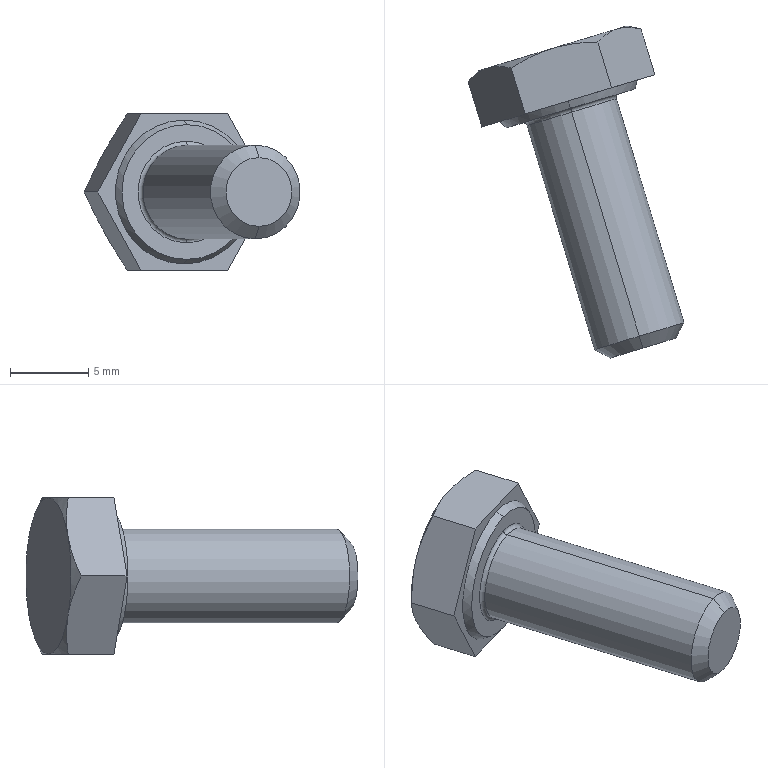Component | SolidWorks | GB_T5781-2000[HexHeadBoltFullThreadGradeCM6_16]-1 | 1 solid | 24 faces | box 13.82 x 21.23 x 10 mm | volume 780 mm3 | cone 10 | plane 10 | cylinder 2 | torus 2 | commonest cylinder face diameters 6 x2
STEP:
#1=COLOUR_RGB('',0.7922,0.8196,0.9333);
#2=FILL_AREA_STYLE_COLOUR('',#1);
#3=FILL_AREA_STYLE('',(#2));
#4=SURFACE_STYLE_FILL_AREA(#3);
#5=SURFACE_SIDE_STYLE('',(#4));
#6=SURFACE_STYLE_USAGE(.BOTH.,#5);
#7=PRESENTATION_STYLE_ASSIGNMENT((#6));
#8=CARTESIAN_POINT('',(-9.837,5.616,-1.85));
#9=VERTEX_POINT('',#8);
#10=CARTESIAN_POINT('',(-9.837,5.616,-2.087));
#11=VERTEX_POINT('',#10);
#12=CARTESIAN_POINT('',(-9.837,5.616,-1.969));
#13=DIRECTION('',(-0.2889,0.9574,0.));
#14=DIRECTION('',(0.,0.,1.));
#15=AXIS2_PLACEMENT_3D('',#12,#13,#14);
#16=CIRCLE('',#15,0.1181);
#17=EDGE_CURVE('',#9,#11,#16,.T.);
#18=ORIENTED_EDGE('',*,*,#17,.F.);
#19=CARTESIAN_POINT('',(-9.667,5.053,-1.85));
#20=VERTEX_POINT('',#19);
#21=CARTESIAN_POINT('',(-9.885,5.776,-1.85));
#22=DIRECTION('',(0.2889,-0.9574,0.));
#23=VECTOR('',#22,39.37);
#24=LINE('',#21,#23);
#25=EDGE_CURVE('',#9,#20,#24,.T.);
#26=ORIENTED_EDGE('',*,*,#25,.T.);
#27=CARTESIAN_POINT('',(-9.667,5.053,-2.087));
#28=VERTEX_POINT('',#27);
#29=CARTESIAN_POINT('',(-9.667,5.053,-1.969));
#30=DIRECTION('',(-0.2889,0.9574,0.));
#31=DIRECTION('',(0.,0.,-1.));
#32=AXIS2_PLACEMENT_3D('',#29,#30,#31);
#33=CIRCLE('',#32,0.1181);
#34=EDGE_CURVE('',#20,#28,#33,.T.);
#35=ORIENTED_EDGE('',*,*,#34,.T.);
#36=CARTESIAN_POINT('',(-9.885,5.776,-2.087));
#37=DIRECTION('',(0.2889,-0.9574,0.));
#38=VECTOR('',#37,39.37);
#39=LINE('',#36,#38);
#40=EDGE_CURVE('',#11,#28,#39,.T.);
#41=ORIENTED_EDGE('',*,*,#40,.F.);
#42=EDGE_LOOP('',(#18,#26,#35,#41));
#43=FACE_OUTER_BOUND('',#42,.T.);
#44=CARTESIAN_POINT('',(-9.885,5.776,-1.969));
#45=DIRECTION('',(0.2889,-0.9574,0.));
#46=DIRECTION('',(0.,0.,-1.));
#47=AXIS2_PLACEMENT_3D('',#44,#45,#46);
#48=CYLINDRICAL_SURFACE('',#47,0.1181);
#49=ADVANCED_FACE('',(#43),#48,.T.);
#50=CARTESIAN_POINT('',(-9.658,5.022,-2.055));
#51=VERTEX_POINT('',#50);
#52=CARTESIAN_POINT('',(-9.658,5.022,-1.882));
#53=VERTEX_POINT('',#52);
#54=CARTESIAN_POINT('',(-9.658,5.022,-1.969));
#55=DIRECTION('',(0.2889,-0.9574,0.));
#56=DIRECTION('',(0.,0.,-1.));
#57=AXIS2_PLACEMENT_3D('',#54,#55,#56);
#58=CIRCLE('',#57,0.08661);
#59=EDGE_CURVE('',#51,#53,#58,.T.);
#60=ORIENTED_EDGE('',*,*,#59,.F.);
#61=CARTESIAN_POINT('',(-9.658,5.022,-2.055));
#62=DIRECTION('',(-0.2043,0.677,-0.7071));
#63=VECTOR('',#62,39.37);
#64=LINE('',#61,#63);
#65=EDGE_CURVE('',#51,#28,#64,.T.);
#66=ORIENTED_EDGE('',*,*,#65,.T.);
#67=ORIENTED_EDGE('',*,*,#34,.F.);
#68=CARTESIAN_POINT('',(-9.658,5.022,-1.882));
#69=DIRECTION('',(-0.2043,0.677,0.7071));
#70=VECTOR('',#69,39.37);
#71=LINE('',#68,#70);
#72=EDGE_CURVE('',#53,#20,#71,.T.);
#73=ORIENTED_EDGE('',*,*,#72,.F.);
#74=EDGE_LOOP('',(#60,#66,#67,#73));
#75=FACE_OUTER_BOUND('',#74,.T.);
#76=CARTESIAN_POINT('',(-9.658,5.022,-1.969));
#77=DIRECTION('',(-0.2889,0.9574,0.));
#78=DIRECTION('',(0.,0.,1.));
#79=AXIS2_PLACEMENT_3D('',#76,#77,#78);
#80=CONICAL_SURFACE('',#79,0.08661,0.7854);
#81=ADVANCED_FACE('',(#75),#80,.T.);
#82=CARTESIAN_POINT('',(-9.84,5.626,-2.096));
#83=VERTEX_POINT('',#82);
#84=CARTESIAN_POINT('',(-9.84,5.626,-1.841));
#85=VERTEX_POINT('',#84);
#86=CARTESIAN_POINT('',(-9.84,5.626,-1.969));
#87=DIRECTION('',(-0.2889,0.9574,0.));
#88=DIRECTION('',(0.,0.,1.));
#89=AXIS2_PLACEMENT_3D('',#86,#87,#88);
#90=CIRCLE('',#89,0.128);
#91=EDGE_CURVE('',#83,#85,#90,.T.);
#92=ORIENTED_EDGE('',*,*,#91,.F.);
#93=CARTESIAN_POINT('',(-9.837,5.616,-2.096));
#94=DIRECTION('',(0.9574,0.2889,0.));
#95=DIRECTION('',(-0.2889,0.9574,0.));
#96=AXIS2_PLACEMENT_3D('',#93,#94,#95);
#97=CIRCLE('',#96,0.009843);
#98=EDGE_CURVE('',#83,#11,#97,.T.);
#99=ORIENTED_EDGE('',*,*,#98,.T.);
#100=CARTESIAN_POINT('',(-9.837,5.616,-1.969));
#101=DIRECTION('',(-0.2889,0.9574,0.));
#102=DIRECTION('',(0.,0.,1.));
#103=AXIS2_PLACEMENT_3D('',#100,#101,#102);
#104=CIRCLE('',#103,0.1181);
#105=EDGE_CURVE('',#11,#9,#104,.T.);
#106=ORIENTED_EDGE('',*,*,#105,.T.);
#107=CARTESIAN_POINT('',(-9.837,5.616,-1.841));
#108=DIRECTION('',(-0.9574,-0.2889,0.));
#109=DIRECTION('',(0.2889,-0.9574,0.));
#110=AXIS2_PLACEMENT_3D('',#107,#108,#109);
#111=CIRCLE('',#110,0.009843);
#112=EDGE_CURVE('',#85,#9,#111,.T.);
#113=ORIENTED_EDGE('',*,*,#112,.F.);
#114=EDGE_LOOP('',(#92,#99,#106,#113));
#115=FACE_OUTER_BOUND('',#114,.T.);
#116=CARTESIAN_POINT('',(-9.837,5.616,-1.969));
#117=DIRECTION('',(-0.2889,0.9574,0.));
#118=DIRECTION('',(0.,0.,1.));
#119=AXIS2_PLACEMENT_3D('',#116,#117,#118);
#120=TOROIDAL_SURFACE('',#119,0.128,0.009843);
#121=ADVANCED_FACE('',(#115),#120,.F.);
#122=CARTESIAN_POINT('',(-9.84,5.626,-1.799));
#123=VERTEX_POINT('',#122);
#124=CARTESIAN_POINT('',(-9.84,5.626,-2.138));
#125=VERTEX_POINT('',#124);
#126=CARTESIAN_POINT('',(-9.84,5.626,-1.969));
#127=DIRECTION('',(-0.2889,0.9574,0.));
#128=DIRECTION('',(0.,0.,1.));
#129=AXIS2_PLACEMENT_3D('',#126,#127,#128);
#130=CIRCLE('',#129,0.1698);
#131=EDGE_CURVE('',#123,#125,#130,.T.);
#132=ORIENTED_EDGE('',*,*,#131,.T.);
#133=CARTESIAN_POINT('',(-9.846,5.644,-2.15));
#134=VERTEX_POINT('',#133);
#135=CARTESIAN_POINT('',(-9.846,5.644,-2.15));
#136=DIRECTION('',(-0.2502,0.8291,-0.5));
#137=VECTOR('',#136,39.37);
#138=LINE('',#135,#137);
#139=EDGE_CURVE('',#125,#134,#138,.T.);
#140=ORIENTED_EDGE('',*,*,#139,.T.);
#141=CARTESIAN_POINT('',(-9.846,5.644,-1.787));
#142=VERTEX_POINT('',#141);
#143=CARTESIAN_POINT('',(-9.846,5.644,-1.969));
#144=DIRECTION('',(-0.2889,0.9574,0.));
#145=DIRECTION('',(0.,0.,1.));
#146=AXIS2_PLACEMENT_3D('',#143,#144,#145);
#147=CIRCLE('',#146,0.1811);
#148=EDGE_CURVE('',#142,#134,#147,.T.);
#149=ORIENTED_EDGE('',*,*,#148,.F.);
#150=CARTESIAN_POINT('',(-9.846,5.644,-1.787));
#151=DIRECTION('',(-0.2502,0.8291,0.5));
#152=VECTOR('',#151,39.37);
#153=LINE('',#150,#152);
#154=EDGE_CURVE('',#123,#142,#153,.T.);
#155=ORIENTED_EDGE('',*,*,#154,.F.);
#156=EDGE_LOOP('',(#132,#140,#149,#155));
#157=FACE_OUTER_BOUND('',#156,.T.);
#158=CARTESIAN_POINT('',(-9.846,5.644,-1.969));
#159=DIRECTION('',(-0.2889,0.9574,0.));
#160=DIRECTION('',(0.,0.,1.));
#161=AXIS2_PLACEMENT_3D('',#158,#159,#160);
#162=CONICAL_SURFACE('',#161,0.1811,0.5236);
#163=ADVANCED_FACE('',(#157),#162,.T.);
#164=ORIENTED_EDGE('',*,*,#131,.F.);
#165=CARTESIAN_POINT('',(-9.84,5.626,-1.969));
#166=DIRECTION('',(-0.2889,0.9574,0.));
#167=DIRECTION('',(0.,0.,1.));
#168=AXIS2_PLACEMENT_3D('',#165,#166,#167);
#169=CIRCLE('',#168,0.1698);
#170=EDGE_CURVE('',#125,#123,#169,.T.);
#171=ORIENTED_EDGE('',*,*,#170,.F.);
#172=EDGE_LOOP('',(#164,#171));
#173=FACE_OUTER_BOUND('',#172,.T.);
#174=CARTESIAN_POINT('',(-9.84,5.626,-1.969));
#175=DIRECTION('',(-0.2889,0.9574,0.));
#176=DIRECTION('',(0.,0.,1.));
#177=AXIS2_PLACEMENT_3D('',#174,#175,#176);
#178=CIRCLE('',#177,0.128);
#179=EDGE_CURVE('',#85,#83,#178,.T.);
#180=ORIENTED_EDGE('',*,*,#179,.T.);
#181=ORIENTED_EDGE('',*,*,#91,.T.);
#182=EDGE_LOOP('',(#180,#181));
#183=FACE_BOUND('',#182,.T.);
#184=CARTESIAN_POINT('',(-9.622,5.691,-1.969));
#185=DIRECTION('',(0.2889,-0.9574,0.));
#186=DIRECTION('',(0.,0.,-1.));
#187=AXIS2_PLACEMENT_3D('',#184,#185,#186);
#188=PLANE('',#187);
#189=ADVANCED_FACE('',(#173,#183),#188,.T.);
#190=CARTESIAN_POINT('',(-9.737,5.677,-2.165));
#191=VERTEX_POINT('',#190);
#192=CARTESIAN_POINT('',(-9.628,5.71,-1.969));
#193=VERTEX_POINT('',#192);
#194=CARTESIAN_POINT('',(-9.737,5.677,-2.165));
#195=DIRECTION('',(0.4787,0.1444,0.866));
#196=VECTOR('',#195,39.37);
#197=LINE('',#194,#196);
#198=EDGE_CURVE('',#191,#193,#197,.T.);
#199=ORIENTED_EDGE('',*,*,#198,.F.);
#200=CARTESIAN_POINT('',(-9.772,5.792,-2.165));
#201=VERTEX_POINT('',#200);
#202=CARTESIAN_POINT('',(-9.731,5.658,-2.165));
#203=DIRECTION('',(-0.2889,0.9574,0.));
#204=VECTOR('',#203,39.37);
#205=LINE('',#202,#204);
#206=EDGE_CURVE('',#191,#201,#205,.T.);
#207=ORIENTED_EDGE('',*,*,#206,.T.);
#208=CARTESIAN_POINT('',(-9.722,5.826,-2.067));
#209=VERTEX_POINT('',#208);
#210=CARTESIAN_POINT('',(-9.722,5.826,-2.067));
#211=CARTESIAN_POINT('',(-9.727,5.824,-2.075));
#212=CARTESIAN_POINT('',(-9.731,5.822,-2.084));
#213=CARTESIAN_POINT('',(-9.74,5.818,-2.1));
#214=CARTESIAN_POINT('',(-9.744,5.816,-2.109));
#215=CARTESIAN_POINT('',(-9.757,5.807,-2.133));
#216=CARTESIAN_POINT('',(-9.764,5.8,-2.149));
#217=CARTESIAN_POINT('',(-9.772,5.792,-2.165));
#218=B_SPLINE_CURVE_WITH_KNOTS('',3,(#210,#211,#212,#213,#214,#215,#216,#217),.UNSPECIFIED.,.F.,.F.,(4,2,2,4),(0.002921,0.003649,0.004376,0.005831),.UNSPECIFIED.);
#219=EDGE_CURVE('',#209,#201,#218,.T.);
#220=ORIENTED_EDGE('',*,*,#219,.F.);
#221=CARTESIAN_POINT('',(-9.663,5.825,-1.969));
#222=VERTEX_POINT('',#221);
#223=CARTESIAN_POINT('',(-9.663,5.825,-1.969));
#224=CARTESIAN_POINT('',(-9.684,5.83,-2.001));
#225=CARTESIAN_POINT('',(-9.704,5.831,-2.033));
#226=CARTESIAN_POINT('',(-9.722,5.826,-2.067));
#227=B_SPLINE_CURVE_WITH_KNOTS('',3,(#223,#224,#225,#226),.UNSPECIFIED.,.F.,.F.,(4,4),(0.00000024,0.002921),.UNSPECIFIED.);
#228=EDGE_CURVE('',#222,#209,#227,.T.);
#229=ORIENTED_EDGE('',*,*,#228,.F.);
#230=CARTESIAN_POINT('',(-9.622,5.691,-1.969));
#231=DIRECTION('',(-0.2889,0.9574,0.));
#232=VECTOR('',#231,39.37);
#233=LINE('',#230,#232);
#234=EDGE_CURVE('',#193,#222,#233,.T.);
#235=ORIENTED_EDGE('',*,*,#234,.F.);
#236=EDGE_LOOP('',(#199,#207,#220,#229,#235));
#237=FACE_OUTER_BOUND('',#236,.T.);
#238=CARTESIAN_POINT('',(-9.731,5.658,-2.165));
#239=DIRECTION('',(-0.8291,-0.2502,0.5));
#240=DIRECTION('',(-0.4787,-0.1444,-0.866));
#241=AXIS2_PLACEMENT_3D('',#238,#239,#240);
#242=PLANE('',#241);
#243=ADVANCED_FACE('',(#237),#242,.F.);
#244=CARTESIAN_POINT('',(-9.737,5.677,-1.772));
#245=VERTEX_POINT('',#244);
#246=CARTESIAN_POINT('',(-9.628,5.71,-1.969));
#247=DIRECTION('',(-0.4787,-0.1444,0.866));
#248=VECTOR('',#247,39.37);
#249=LINE('',#246,#248);
#250=EDGE_CURVE('',#193,#245,#249,.T.);
#251=ORIENTED_EDGE('',*,*,#250,.F.);
#252=ORIENTED_EDGE('',*,*,#234,.T.);
#253=CARTESIAN_POINT('',(-9.722,5.826,-1.87));
#254=VERTEX_POINT('',#253);
#255=CARTESIAN_POINT('',(-9.722,5.826,-1.87));
#256=CARTESIAN_POINT('',(-9.718,5.827,-1.878));
#257=CARTESIAN_POINT('',(-9.713,5.828,-1.887));
#258=CARTESIAN_POINT('',(-9.703,5.829,-1.903));
#259=CARTESIAN_POINT('',(-9.698,5.829,-1.912));
#260=CARTESIAN_POINT('',(-9.683,5.829,-1.936));
#261=CARTESIAN_POINT('',(-9.673,5.828,-1.952));
#262=CARTESIAN_POINT('',(-9.663,5.825,-1.969));
#263=B_SPLINE_CURVE_WITH_KNOTS('',3,(#255,#256,#257,#258,#259,#260,#261,#262),.UNSPECIFIED.,.F.,.F.,(4,2,2,4),(0.002921,0.003649,0.004376,0.005831),.UNSPECIFIED.);
#264=EDGE_CURVE('',#254,#222,#263,.T.);
#265=ORIENTED_EDGE('',*,*,#264,.F.);
#266=CARTESIAN_POINT('',(-9.772,5.792,-1.772));
#267=VERTEX_POINT('',#266);
#268=CARTESIAN_POINT('',(-9.772,5.792,-1.772));
#269=CARTESIAN_POINT('',(-9.757,5.808,-1.804));
#270=CARTESIAN_POINT('',(-9.741,5.82,-1.837));
#271=CARTESIAN_POINT('',(-9.722,5.826,-1.87));
#272=B_SPLINE_CURVE_WITH_KNOTS('',3,(#268,#269,#270,#271),.UNSPECIFIED.,.F.,.F.,(4,4),(0.00000024,0.002921),.UNSPECIFIED.);
#273=EDGE_CURVE('',#267,#254,#272,.T.);
#274=ORIENTED_EDGE('',*,*,#273,.F.);
#275=CARTESIAN_POINT('',(-9.731,5.658,-1.772));
#276=DIRECTION('',(-0.2889,0.9574,0.));
#277=VECTOR('',#276,39.37);
#278=LINE('',#275,#277);
#279=EDGE_CURVE('',#245,#267,#278,.T.);
#280=ORIENTED_EDGE('',*,*,#279,.F.);
#281=EDGE_LOOP('',(#251,#252,#265,#274,#280));
#282=FACE_OUTER_BOUND('',#281,.T.);
#283=CARTESIAN_POINT('',(-9.622,5.691,-1.969));
#284=DIRECTION('',(-0.8291,-0.2502,-0.5));
#285=DIRECTION('',(0.4787,0.1444,-0.866));
#286=AXIS2_PLACEMENT_3D('',#283,#284,#285);
#287=PLANE('',#286);
#288=ADVANCED_FACE('',(#282),#287,.F.);
#289=CARTESIAN_POINT('',(-9.954,5.612,-1.772));
#290=VERTEX_POINT('',#289);
#291=CARTESIAN_POINT('',(-9.737,5.677,-1.772));
#292=DIRECTION('',(-0.9574,-0.2889,-0.));
#293=VECTOR('',#292,39.37);
#294=LINE('',#291,#293);
#295=EDGE_CURVE('',#245,#290,#294,.T.);
#296=ORIENTED_EDGE('',*,*,#295,.F.);
#297=ORIENTED_EDGE('',*,*,#279,.T.);
#298=CARTESIAN_POINT('',(-9.885,5.776,-1.772));
#299=VERTEX_POINT('',#298);
#300=CARTESIAN_POINT('',(-9.885,5.776,-1.772));
#301=CARTESIAN_POINT('',(-9.867,5.782,-1.772));
#302=CARTESIAN_POINT('',(-9.848,5.786,-1.772));
#303=CARTESIAN_POINT('',(-9.81,5.791,-1.772));
#304=CARTESIAN_POINT('',(-9.791,5.792,-1.772));
#305=CARTESIAN_POINT('',(-9.772,5.792,-1.772));
#306=B_SPLINE_CURVE_WITH_KNOTS('',3,(#300,#301,#302,#303,#304,#305),.UNSPECIFIED.,.F.,.F.,(4,2,4),(0.008262,0.009724,0.01119),.UNSPECIFIED.);
#307=EDGE_CURVE('',#299,#267,#306,.T.);
#308=ORIENTED_EDGE('',*,*,#307,.F.);
#309=CARTESIAN_POINT('',(-9.989,5.727,-1.772));
#310=VERTEX_POINT('',#309);
#311=CARTESIAN_POINT('',(-9.989,5.727,-1.772));
#312=CARTESIAN_POINT('',(-9.973,5.737,-1.772));
#313=CARTESIAN_POINT('',(-9.956,5.747,-1.772));
#314=CARTESIAN_POINT('',(-9.922,5.764,-1.772));
#315=CARTESIAN_POINT('',(-9.904,5.771,-1.772));
#316=CARTESIAN_POINT('',(-9.885,5.776,-1.772));
#317=B_SPLINE_CURVE_WITH_KNOTS('',3,(#311,#312,#313,#314,#315,#316),.UNSPECIFIED.,.F.,.F.,(4,2,4),(0.00534,0.006801,0.008262),.UNSPECIFIED.);
#318=EDGE_CURVE('',#310,#299,#317,.T.);
#319=ORIENTED_EDGE('',*,*,#318,.F.);
#320=CARTESIAN_POINT('',(-9.949,5.593,-1.772));
#321=DIRECTION('',(-0.2889,0.9574,0.));
#322=VECTOR('',#321,39.37);
#323=LINE('',#320,#322);
#324=EDGE_CURVE('',#290,#310,#323,.T.);
#325=ORIENTED_EDGE('',*,*,#324,.F.);
#326=EDGE_LOOP('',(#296,#297,#308,#319,#325));
#327=FACE_OUTER_BOUND('',#326,.T.);
#328=CARTESIAN_POINT('',(-9.731,5.658,-1.772));
#329=DIRECTION('',(0.,0.,-1.));
#330=DIRECTION('',(0.9574,0.2889,0.));
#331=AXIS2_PLACEMENT_3D('',#328,#329,#330);
#332=PLANE('',#331);
#333=ADVANCED_FACE('',(#327),#332,.F.);
#334=CARTESIAN_POINT('',(-10.063,5.579,-1.969));
#335=VERTEX_POINT('',#334);
#336=CARTESIAN_POINT('',(-10.063,5.579,-1.969));
#337=DIRECTION('',(-0.4787,-0.1444,-0.866));
#338=VECTOR('',#337,39.37);
#339=LINE('',#336,#338);
#340=EDGE_CURVE('',#290,#335,#339,.T.);
#341=ORIENTED_EDGE('',*,*,#340,.F.);
#342=ORIENTED_EDGE('',*,*,#324,.T.);
#343=CARTESIAN_POINT('',(-10.049,5.727,-1.87));
#344=VERTEX_POINT('',#343);
#345=CARTESIAN_POINT('',(-10.049,5.727,-1.87));
#346=CARTESIAN_POINT('',(-10.044,5.728,-1.862));
#347=CARTESIAN_POINT('',(-10.039,5.729,-1.853));
#348=CARTESIAN_POINT('',(-10.03,5.731,-1.837));
#349=CARTESIAN_POINT('',(-10.025,5.731,-1.828));
#350=CARTESIAN_POINT('',(-10.01,5.731,-1.804));
#351=CARTESIAN_POINT('',(-10.,5.729,-1.788));
#352=CARTESIAN_POINT('',(-9.989,5.727,-1.772));
#353=B_SPLINE_CURVE_WITH_KNOTS('',3,(#345,#346,#347,#348,#349,#350,#351,#352),.UNSPECIFIED.,.F.,.F.,(4,2,2,4),(0.002921,0.003649,0.004376,0.005831),.UNSPECIFIED.);
#354=EDGE_CURVE('',#344,#310,#353,.T.);
#355=ORIENTED_EDGE('',*,*,#354,.F.);
#356=CARTESIAN_POINT('',(-10.098,5.694,-1.969));
#357=VERTEX_POINT('',#356);
#358=CARTESIAN_POINT('',(-10.098,5.694,-1.969));
#359=CARTESIAN_POINT('',(-10.083,5.709,-1.936));
#360=CARTESIAN_POINT('',(-10.067,5.721,-1.904));
#361=CARTESIAN_POINT('',(-10.049,5.727,-1.87));
#362=B_SPLINE_CURVE_WITH_KNOTS('',3,(#358,#359,#360,#361),.UNSPECIFIED.,.F.,.F.,(4,4),(0.00000024,0.002921),.UNSPECIFIED.);
#363=EDGE_CURVE('',#357,#344,#362,.T.);
#364=ORIENTED_EDGE('',*,*,#363,.F.);
#365=CARTESIAN_POINT('',(-10.058,5.56,-1.969));
#366=DIRECTION('',(-0.2889,0.9574,0.));
#367=VECTOR('',#366,39.37);
#368=LINE('',#365,#367);
#369=EDGE_CURVE('',#335,#357,#368,.T.);
#370=ORIENTED_EDGE('',*,*,#369,.F.);
#371=EDGE_LOOP('',(#341,#342,#355,#364,#370));
#372=FACE_OUTER_BOUND('',#371,.T.);
#373=CARTESIAN_POINT('',(-10.058,5.56,-1.969));
#374=DIRECTION('',(0.8291,0.2502,-0.5));
#375=DIRECTION('',(0.4787,0.1444,0.866));
#376=AXIS2_PLACEMENT_3D('',#373,#374,#375);
#377=PLANE('',#376);
#378=ADVANCED_FACE('',(#372),#377,.F.);
#379=CARTESIAN_POINT('',(-9.954,5.612,-2.165));
#380=VERTEX_POINT('',#379);
#381=CARTESIAN_POINT('',(-9.954,5.612,-2.165));
#382=DIRECTION('',(0.4787,0.1444,-0.866));
#383=VECTOR('',#382,39.37);
#384=LINE('',#381,#383);
#385=EDGE_CURVE('',#335,#380,#384,.T.);
#386=ORIENTED_EDGE('',*,*,#385,.F.);
#387=ORIENTED_EDGE('',*,*,#369,.T.);
#388=CARTESIAN_POINT('',(-10.049,5.727,-2.067));
#389=VERTEX_POINT('',#388);
#390=CARTESIAN_POINT('',(-10.049,5.727,-2.067));
#391=CARTESIAN_POINT('',(-10.053,5.726,-2.059));
#392=CARTESIAN_POINT('',(-10.058,5.724,-2.05));
#393=CARTESIAN_POINT('',(-10.067,5.72,-2.034));
#394=CARTESIAN_POINT('',(-10.071,5.717,-2.025));
#395=CARTESIAN_POINT('',(-10.083,5.709,-2.001));
#396=CARTESIAN_POINT('',(-10.091,5.702,-1.985));
#397=CARTESIAN_POINT('',(-10.098,5.694,-1.969));
#398=B_SPLINE_CURVE_WITH_KNOTS('',3,(#390,#391,#392,#393,#394,#395,#396,#397),.UNSPECIFIED.,.F.,.F.,(4,2,2,4),(0.002921,0.003649,0.004376,0.005831),.UNSPECIFIED.);
#399=EDGE_CURVE('',#389,#357,#398,.T.);
#400=ORIENTED_EDGE('',*,*,#399,.F.);
#401=CARTESIAN_POINT('',(-9.989,5.727,-2.165));
#402=VERTEX_POINT('',#401);
#403=CARTESIAN_POINT('',(-9.989,5.727,-2.165));
#404=CARTESIAN_POINT('',(-10.01,5.732,-2.133));
#405=CARTESIAN_POINT('',(-10.03,5.733,-2.1));
#406=CARTESIAN_POINT('',(-10.049,5.727,-2.067));
#407=B_SPLINE_CURVE_WITH_KNOTS('',3,(#403,#404,#405,#406),.UNSPECIFIED.,.F.,.F.,(4,4),(0.00000024,0.002921),.UNSPECIFIED.);
#408=EDGE_CURVE('',#402,#389,#407,.T.);
#409=ORIENTED_EDGE('',*,*,#408,.F.);
#410=CARTESIAN_POINT('',(-9.949,5.593,-2.165));
#411=DIRECTION('',(-0.2889,0.9574,0.));
#412=VECTOR('',#411,39.37);
#413=LINE('',#410,#412);
#414=EDGE_CURVE('',#380,#402,#413,.T.);
#415=ORIENTED_EDGE('',*,*,#414,.F.);
#416=EDGE_LOOP('',(#386,#387,#400,#409,#415));
#417=FACE_OUTER_BOUND('',#416,.T.);
#418=CARTESIAN_POINT('',(-9.949,5.593,-2.165));
#419=DIRECTION('',(0.8291,0.2502,0.5));
#420=DIRECTION('',(-0.4787,-0.1444,0.866));
#421=AXIS2_PLACEMENT_3D('',#418,#419,#420);
#422=PLANE('',#421);
#423=ADVANCED_FACE('',(#417),#422,.F.);
#424=CARTESIAN_POINT('',(-9.737,5.677,-2.165));
#425=DIRECTION('',(0.9574,0.2889,0.));
#426=VECTOR('',#425,39.37);
#427=LINE('',#424,#426);
#428=EDGE_CURVE('',#380,#191,#427,.T.);
#429=ORIENTED_EDGE('',*,*,#428,.F.);
#430=ORIENTED_EDGE('',*,*,#414,.T.);
#431=CARTESIAN_POINT('',(-9.885,5.776,-2.165));
#432=VERTEX_POINT('',#431);
#433=CARTESIAN_POINT('',(-9.885,5.776,-2.165));
#434=CARTESIAN_POINT('',(-9.904,5.771,-2.165));
#435=CARTESIAN_POINT('',(-9.922,5.764,-2.165));
#436=CARTESIAN_POINT('',(-9.956,5.747,-2.165));
#437=CARTESIAN_POINT('',(-9.973,5.737,-2.165));
#438=CARTESIAN_POINT('',(-9.989,5.727,-2.165));
#439=B_SPLINE_CURVE_WITH_KNOTS('',3,(#433,#434,#435,#436,#437,#438),.UNSPECIFIED.,.F.,.F.,(4,2,4),(0.01799,0.01945,0.02091),.UNSPECIFIED.);
#440=EDGE_CURVE('',#432,#402,#439,.T.);
#441=ORIENTED_EDGE('',*,*,#440,.F.);
#442=CARTESIAN_POINT('',(-9.772,5.792,-2.165));
#443=CARTESIAN_POINT('',(-9.791,5.792,-2.165));
#444=CARTESIAN_POINT('',(-9.81,5.791,-2.165));
#445=CARTESIAN_POINT('',(-9.848,5.786,-2.165));
#446=CARTESIAN_POINT('',(-9.867,5.782,-2.165));
#447=CARTESIAN_POINT('',(-9.885,5.776,-2.165));
#448=B_SPLINE_CURVE_WITH_KNOTS('',3,(#442,#443,#444,#445,#446,#447),.UNSPECIFIED.,.F.,.F.,(4,2,4),(0.01507,0.01653,0.01799),.UNSPECIFIED.);
#449=EDGE_CURVE('',#201,#432,#448,.T.);
#450=ORIENTED_EDGE('',*,*,#449,.F.);
#451=ORIENTED_EDGE('',*,*,#206,.F.);
#452=EDGE_LOOP('',(#429,#430,#441,#450,#451));
#453=FACE_OUTER_BOUND('',#452,.T.);
#454=CARTESIAN_POINT('',(-9.731,5.658,-2.165));
#455=DIRECTION('',(0.,0.,1.));
#456=DIRECTION('',(0.2889,-0.9574,0.));
#457=AXIS2_PLACEMENT_3D('',#454,#455,#456);
#458=PLANE('',#457);
#459=ADVANCED_FACE('',(#453),#458,.F.);
#460=ORIENTED_EDGE('',*,*,#408,.T.);
#461=CARTESIAN_POINT('',(-9.885,5.776,-1.969));
#462=DIRECTION('',(0.2889,-0.9574,0.));
#463=DIRECTION('',(0.,0.,-1.));
#464=AXIS2_PLACEMENT_3D('',#461,#462,#463);
#465=CIRCLE('',#464,0.1969);
#466=EDGE_CURVE('',#389,#432,#465,.T.);
#467=ORIENTED_EDGE('',*,*,#466,.T.);
#468=ORIENTED_EDGE('',*,*,#440,.T.);
#469=EDGE_LOOP('',(#460,#467,#468));
#470=FACE_OUTER_BOUND('',#469,.T.);
#471=CARTESIAN_POINT('',(-9.885,5.776,-1.969));
#472=DIRECTION('',(0.2889,-0.9574,0.));
#473=DIRECTION('',(0.,0.,-1.));
#474=AXIS2_PLACEMENT_3D('',#471,#472,#473);
#475=CONICAL_SURFACE('',#474,0.1969,1.047);
#476=ADVANCED_FACE('',(#470),#475,.T.);
#477=ORIENTED_EDGE('',*,*,#363,.T.);
#478=CARTESIAN_POINT('',(-9.885,5.776,-1.969));
#479=DIRECTION('',(0.2889,-0.9574,0.));
#480=DIRECTION('',(0.,0.,-1.));
#481=AXIS2_PLACEMENT_3D('',#478,#479,#480);
#482=CIRCLE('',#481,0.1969);
#483=EDGE_CURVE('',#344,#389,#482,.T.);
#484=ORIENTED_EDGE('',*,*,#483,.T.);
#485=ORIENTED_EDGE('',*,*,#399,.T.);
#486=EDGE_LOOP('',(#477,#484,#485));
#487=FACE_OUTER_BOUND('',#486,.T.);
#488=CARTESIAN_POINT('',(-9.885,5.776,-1.969));
#489=DIRECTION('',(0.2889,-0.9574,0.));
#490=DIRECTION('',(0.,0.,-1.));
#491=AXIS2_PLACEMENT_3D('',#488,#489,#490);
#492=CONICAL_SURFACE('',#491,0.1969,1.047);
#493=ADVANCED_FACE('',(#487),#492,.T.);
#494=ORIENTED_EDGE('',*,*,#318,.T.);
#495=CARTESIAN_POINT('',(-9.885,5.776,-1.969));
#496=DIRECTION('',(0.2889,-0.9574,0.));
#497=DIRECTION('',(0.,0.,-1.));
#498=AXIS2_PLACEMENT_3D('',#495,#496,#497);
#499=CIRCLE('',#498,0.1969);
#500=EDGE_CURVE('',#299,#344,#499,.T.);
#501=ORIENTED_EDGE('',*,*,#500,.T.);
#502=ORIENTED_EDGE('',*,*,#354,.T.);
#503=EDGE_LOOP('',(#494,#501,#502));
#504=FACE_OUTER_BOUND('',#503,.T.);
#505=CARTESIAN_POINT('',(-9.885,5.776,-1.969));
#506=DIRECTION('',(0.2889,-0.9574,0.));
#507=DIRECTION('',(0.,0.,-1.));
#508=AXIS2_PLACEMENT_3D('',#505,#506,#507);
#509=CONICAL_SURFACE('',#508,0.1969,1.047);
#510=ADVANCED_FACE('',(#504),#509,.T.);
#511=ORIENTED_EDGE('',*,*,#307,.T.);
#512=ORIENTED_EDGE('',*,*,#273,.T.);
#513=CARTESIAN_POINT('',(-9.885,5.776,-1.969));
#514=DIRECTION('',(-0.2889,0.9574,0.));
#515=DIRECTION('',(0.,0.,1.));
#516=AXIS2_PLACEMENT_3D('',#513,#514,#515);
#517=CIRCLE('',#516,0.1969);
#518=EDGE_CURVE('',#299,#254,#517,.T.);
#519=ORIENTED_EDGE('',*,*,#518,.F.);
#520=EDGE_LOOP('',(#511,#512,#519));
#521=FACE_OUTER_BOUND('',#520,.T.);
#522=CARTESIAN_POINT('',(-9.885,5.776,-1.969));
#523=DIRECTION('',(0.2889,-0.9574,0.));
#524=DIRECTION('',(0.,0.,-1.));
#525=AXIS2_PLACEMENT_3D('',#522,#523,#524);
#526=CONICAL_SURFACE('',#525,0.1969,1.047);
#527=ADVANCED_FACE('',(#521),#526,.T.);
#528=ORIENTED_EDGE('',*,*,#264,.T.);
#529=ORIENTED_EDGE('',*,*,#228,.T.);
#530=CARTESIAN_POINT('',(-9.885,5.776,-1.969));
#531=DIRECTION('',(0.2889,-0.9574,0.));
#532=DIRECTION('',(0.,0.,-1.));
#533=AXIS2_PLACEMENT_3D('',#530,#531,#532);
#534=CIRCLE('',#533,0.1969);
#535=EDGE_CURVE('',#209,#254,#534,.T.);
#536=ORIENTED_EDGE('',*,*,#535,.T.);
#537=EDGE_LOOP('',(#528,#529,#536));
#538=FACE_OUTER_BOUND('',#537,.T.);
#539=CARTESIAN_POINT('',(-9.885,5.776,-1.969));
#540=DIRECTION('',(0.2889,-0.9574,0.));
#541=DIRECTION('',(0.,0.,-1.));
#542=AXIS2_PLACEMENT_3D('',#539,#540,#541);
#543=CONICAL_SURFACE('',#542,0.1969,1.047);
#544=ADVANCED_FACE('',(#538),#543,.T.);
#545=ORIENTED_EDGE('',*,*,#219,.T.);
#546=ORIENTED_EDGE('',*,*,#449,.T.);
#547=CARTESIAN_POINT('',(-9.885,5.776,-1.969));
#548=DIRECTION('',(0.2889,-0.9574,0.));
#549=DIRECTION('',(0.,0.,-1.));
#550=AXIS2_PLACEMENT_3D('',#547,#548,#549);
#551=CIRCLE('',#550,0.1969);
#552=EDGE_CURVE('',#432,#209,#551,.T.);
#553=ORIENTED_EDGE('',*,*,#552,.T.);
#554=EDGE_LOOP('',(#545,#546,#553));
#555=FACE_OUTER_BOUND('',#554,.T.);
#556=CARTESIAN_POINT('',(-9.885,5.776,-1.969));
#557=DIRECTION('',(0.2889,-0.9574,0.));
#558=DIRECTION('',(0.,0.,-1.));
#559=AXIS2_PLACEMENT_3D('',#556,#557,#558);
#560=CONICAL_SURFACE('',#559,0.1969,1.047);
#561=ADVANCED_FACE('',(#555),#560,.T.);
#562=ORIENTED_EDGE('',*,*,#552,.F.);
#563=ORIENTED_EDGE('',*,*,#466,.F.);
#564=ORIENTED_EDGE('',*,*,#483,.F.);
#565=ORIENTED_EDGE('',*,*,#500,.F.);
#566=ORIENTED_EDGE('',*,*,#518,.T.);
#567=ORIENTED_EDGE('',*,*,#535,.F.);
#568=EDGE_LOOP('',(#562,#563,#564,#565,#566,#567));
#569=FACE_OUTER_BOUND('',#568,.T.);
#570=CARTESIAN_POINT('',(-9.668,5.842,-1.969));
#571=DIRECTION('',(0.2889,-0.9574,0.));
#572=DIRECTION('',(0.,0.,-1.));
#573=AXIS2_PLACEMENT_3D('',#570,#571,#572);
#574=PLANE('',#573);
#575=ADVANCED_FACE('',(#569),#574,.F.);
#576=ORIENTED_EDGE('',*,*,#148,.T.);
#577=CARTESIAN_POINT('',(-9.846,5.644,-1.969));
#578=DIRECTION('',(-0.2889,0.9574,0.));
#579=DIRECTION('',(0.,0.,1.));
#580=AXIS2_PLACEMENT_3D('',#577,#578,#579);
#581=CIRCLE('',#580,0.1811);
#582=EDGE_CURVE('',#134,#142,#581,.T.);
#583=ORIENTED_EDGE('',*,*,#582,.T.);
#584=EDGE_LOOP('',(#576,#583));
#585=FACE_BOUND('',#584,.T.);
#586=ORIENTED_EDGE('',*,*,#198,.T.);
#587=ORIENTED_EDGE('',*,*,#250,.T.);
#588=ORIENTED_EDGE('',*,*,#295,.T.);
#589=ORIENTED_EDGE('',*,*,#340,.T.);
#590=ORIENTED_EDGE('',*,*,#385,.T.);
#591=ORIENTED_EDGE('',*,*,#428,.T.);
#592=EDGE_LOOP('',(#586,#587,#588,#589,#590,#591));
#593=FACE_OUTER_BOUND('',#592,.T.);
#594=CARTESIAN_POINT('',(-9.672,5.697,-1.969));
#595=DIRECTION('',(0.2889,-0.9574,0.));
#596=DIRECTION('',(0.,0.,-1.));
#597=AXIS2_PLACEMENT_3D('',#594,#595,#596);
#598=PLANE('',#597);
#599=ADVANCED_FACE('',(#585,#593),#598,.T.);
#600=ORIENTED_EDGE('',*,*,#139,.F.);
#601=ORIENTED_EDGE('',*,*,#170,.T.);
#602=ORIENTED_EDGE('',*,*,#154,.T.);
#603=ORIENTED_EDGE('',*,*,#582,.F.);
#604=EDGE_LOOP('',(#600,#601,#602,#603));
#605=FACE_OUTER_BOUND('',#604,.T.);
#606=CARTESIAN_POINT('',(-9.846,5.644,-1.969));
#607=DIRECTION('',(-0.2889,0.9574,0.));
#608=DIRECTION('',(0.,0.,1.));
#609=AXIS2_PLACEMENT_3D('',#606,#607,#608);
#610=CONICAL_SURFACE('',#609,0.1811,0.5236);
#611=ADVANCED_FACE('',(#605),#610,.T.);
#612=ORIENTED_EDGE('',*,*,#98,.F.);
#613=ORIENTED_EDGE('',*,*,#179,.F.);
#614=ORIENTED_EDGE('',*,*,#112,.T.);
#615=ORIENTED_EDGE('',*,*,#17,.T.);
#616=EDGE_LOOP('',(#612,#613,#614,#615));
#617=FACE_OUTER_BOUND('',#616,.T.);
#618=CARTESIAN_POINT('',(-9.837,5.616,-1.969));
#619=DIRECTION('',(-0.2889,0.9574,0.));
#620=DIRECTION('',(0.,0.,1.));
#621=AXIS2_PLACEMENT_3D('',#618,#619,#620);
#622=TOROIDAL_SURFACE('',#621,0.128,0.009843);
#623=ADVANCED_FACE('',(#617),#622,.F.);
#624=CARTESIAN_POINT('',(-9.658,5.022,-1.969));
#625=DIRECTION('',(0.2889,-0.9574,0.));
#626=DIRECTION('',(0.,0.,-1.));
#627=AXIS2_PLACEMENT_3D('',#624,#625,#626);
#628=CIRCLE('',#627,0.08661);
#629=EDGE_CURVE('',#53,#51,#628,.T.);
#630=ORIENTED_EDGE('',*,*,#629,.T.);
#631=ORIENTED_EDGE('',*,*,#59,.T.);
#632=EDGE_LOOP('',(#630,#631));
#633=FACE_OUTER_BOUND('',#632,.T.);
#634=CARTESIAN_POINT('',(-9.658,5.022,-1.969));
#635=DIRECTION('',(0.2889,-0.9574,0.));
#636=DIRECTION('',(0.,0.,-1.));
#637=AXIS2_PLACEMENT_3D('',#634,#635,#636);
#638=PLANE('',#637);
#639=ADVANCED_FACE('',(#633),#638,.T.);
#640=ORIENTED_EDGE('',*,*,#65,.F.);
#641=ORIENTED_EDGE('',*,*,#629,.F.);
#642=ORIENTED_EDGE('',*,*,#72,.T.);
#643=CARTESIAN_POINT('',(-9.667,5.053,-1.969));
#644=DIRECTION('',(-0.2889,0.9574,0.));
#645=DIRECTION('',(-0.,0.,-1.));
#646=AXIS2_PLACEMENT_3D('',#643,#644,#645);
#647=CIRCLE('',#646,0.1181);
#648=EDGE_CURVE('',#28,#20,#647,.T.);
#649=ORIENTED_EDGE('',*,*,#648,.F.);
#650=EDGE_LOOP('',(#640,#641,#642,#649));
#651=FACE_OUTER_BOUND('',#650,.T.);
#652=CARTESIAN_POINT('',(-9.658,5.022,-1.969));
#653=DIRECTION('',(-0.2889,0.9574,0.));
#654=DIRECTION('',(0.,0.,1.));
#655=AXIS2_PLACEMENT_3D('',#652,#653,#654);
#656=CONICAL_SURFACE('',#655,0.08661,0.7854);
#657=ADVANCED_FACE('',(#651),#656,.T.);
#658=ORIENTED_EDGE('',*,*,#25,.F.);
#659=ORIENTED_EDGE('',*,*,#105,.F.);
#660=ORIENTED_EDGE('',*,*,#40,.T.);
#661=ORIENTED_EDGE('',*,*,#648,.T.);
#662=EDGE_LOOP('',(#658,#659,#660,#661));
#663=FACE_OUTER_BOUND('',#662,.T.);
#664=CARTESIAN_POINT('',(-9.885,5.776,-1.969));
#665=DIRECTION('',(0.2889,-0.9574,0.));
#666=DIRECTION('',(0.,0.,-1.));
#667=AXIS2_PLACEMENT_3D('',#664,#665,#666);
#668=CYLINDRICAL_SURFACE('',#667,0.1181);
#669=ADVANCED_FACE('',(#663),#668,.T.);
#670=CLOSED_SHELL('',(#49,#81,#121,#163,#189,#243,#288,#333,#378,#423,#459,#476,#493,#510,#527,#544,#561,#575,#599,#611,#623,#639,#657,#669));
#671=MANIFOLD_SOLID_BREP('',#670);
#672=STYLED_ITEM('',(#7),#671);
#673=PRESENTATION_LAYER_ASSIGNMENT('','',(#672));
#674=(LENGTH_UNIT()NAMED_UNIT(*)SI_UNIT($,.METRE.));
#675=LENGTH_MEASURE_WITH_UNIT(LENGTH_MEASURE(0.0254),#674);
#676=DIMENSIONAL_EXPONENTS(1.,0.,0.,0.,0.,0.,0.);
#677=(CONVERSION_BASED_UNIT('',#675)LENGTH_UNIT()NAMED_UNIT(#676));
#678=UNCERTAINTY_MEASURE_WITH_UNIT(LENGTH_MEASURE(0.00001),#677,'','');
#679=(NAMED_UNIT(*)PLANE_ANGLE_UNIT()SI_UNIT($,.RADIAN.));
#680=(NAMED_UNIT(*)SI_UNIT($,.STERADIAN.)SOLID_ANGLE_UNIT());
#681=(GEOMETRIC_REPRESENTATION_CONTEXT(3)GLOBAL_UNCERTAINTY_ASSIGNED_CONTEXT((#678))GLOBAL_UNIT_ASSIGNED_CONTEXT((#677,#679,#680))REPRESENTATION_CONTEXT('',''));
#682=MECHANICAL_DESIGN_GEOMETRIC_PRESENTATION_REPRESENTATION('',(#672),#681);
#683=CARTESIAN_POINT('',(0.,0.,0.));
#684=DIRECTION('',(0.,0.,1.));
#685=DIRECTION('',(1.,0.,0.));
#686=AXIS2_PLACEMENT_3D('',#683,#684,#685);
#687=(LENGTH_UNIT()NAMED_UNIT(*)SI_UNIT($,.METRE.));
#688=LENGTH_MEASURE_WITH_UNIT(LENGTH_MEASURE(0.0254),#687);
#689=DIMENSIONAL_EXPONENTS(1.,0.,0.,0.,0.,0.,0.);
#690=(CONVERSION_BASED_UNIT('',#688)LENGTH_UNIT()NAMED_UNIT(#689));
#691=UNCERTAINTY_MEASURE_WITH_UNIT(LENGTH_MEASURE(0.00001),#690,'','');
#692=(NAMED_UNIT(*)PLANE_ANGLE_UNIT()SI_UNIT($,.RADIAN.));
#693=(NAMED_UNIT(*)SI_UNIT($,.STERADIAN.)SOLID_ANGLE_UNIT());
#694=(GEOMETRIC_REPRESENTATION_CONTEXT(3)GLOBAL_UNCERTAINTY_ASSIGNED_CONTEXT((#691))GLOBAL_UNIT_ASSIGNED_CONTEXT((#690,#692,#693))REPRESENTATION_CONTEXT('',''));
#695=ADVANCED_BREP_SHAPE_REPRESENTATION('',(#671,#686),#694);